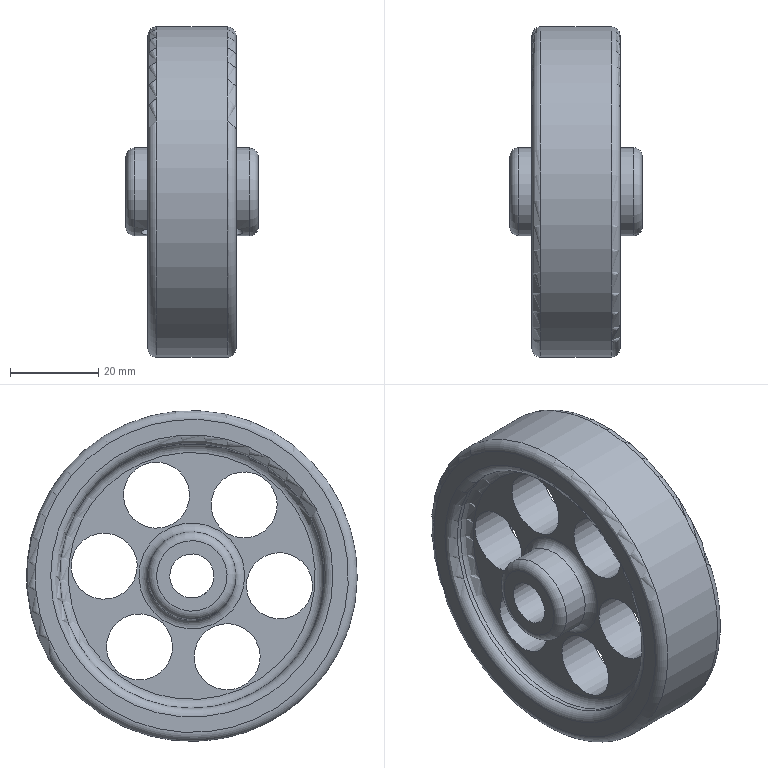Component | NX | 19__27 | 1 solid | 30 faces | volume 52934 mm3 | cylinder 14 | torus 10 | plane 6 | commonest cylinder face diameters 15 x6 20 x2 60 x2 3 x2 10 x1 75 x1